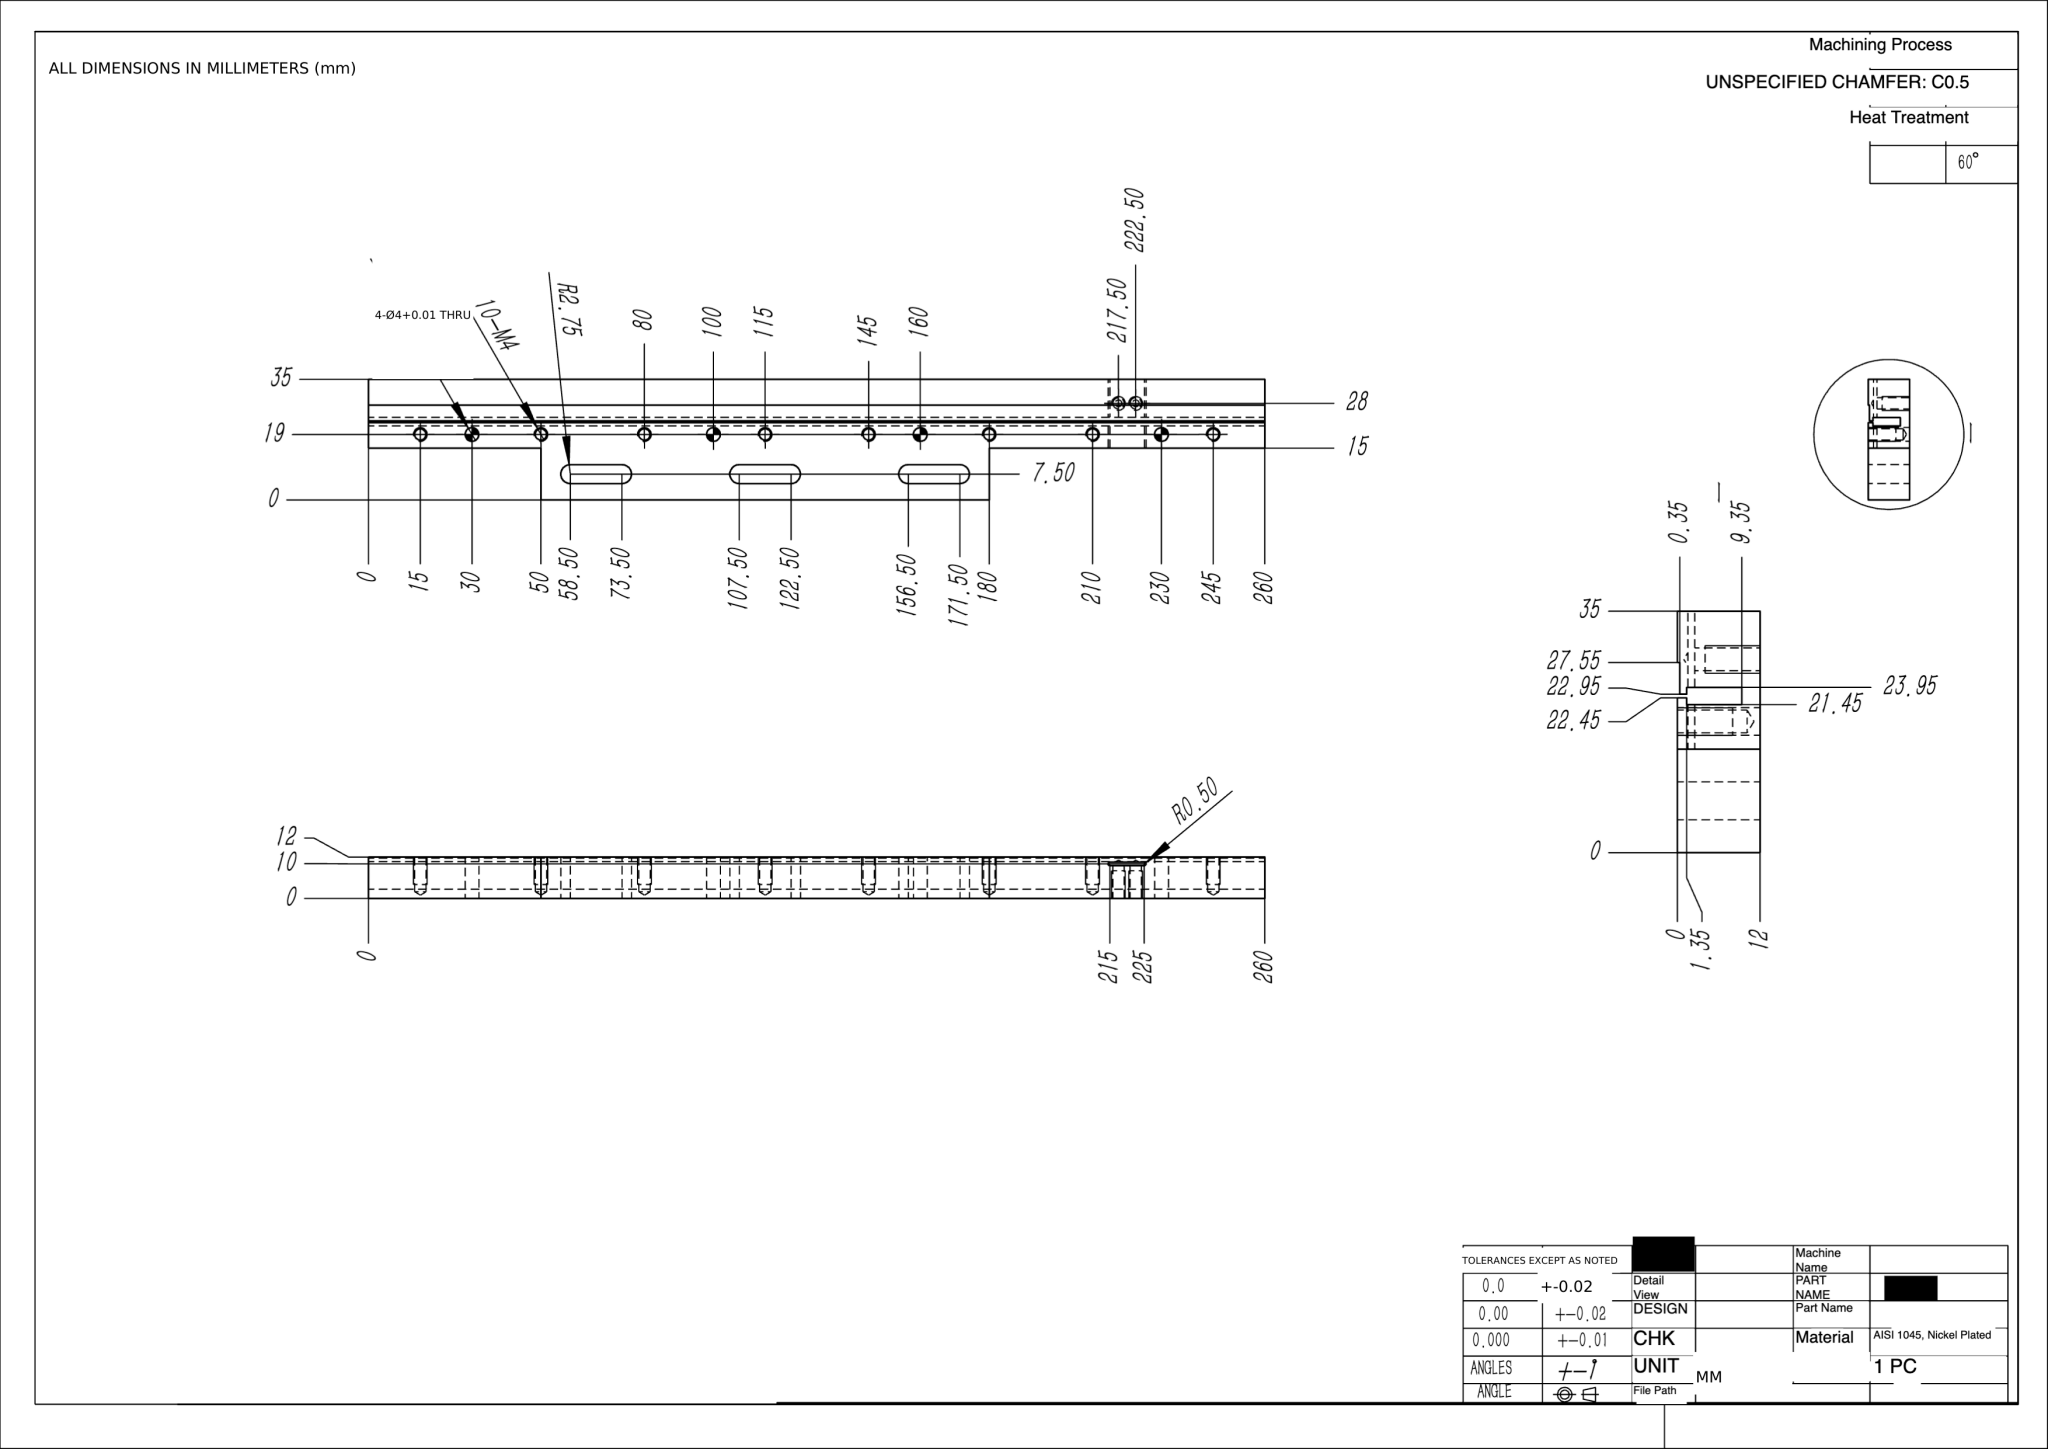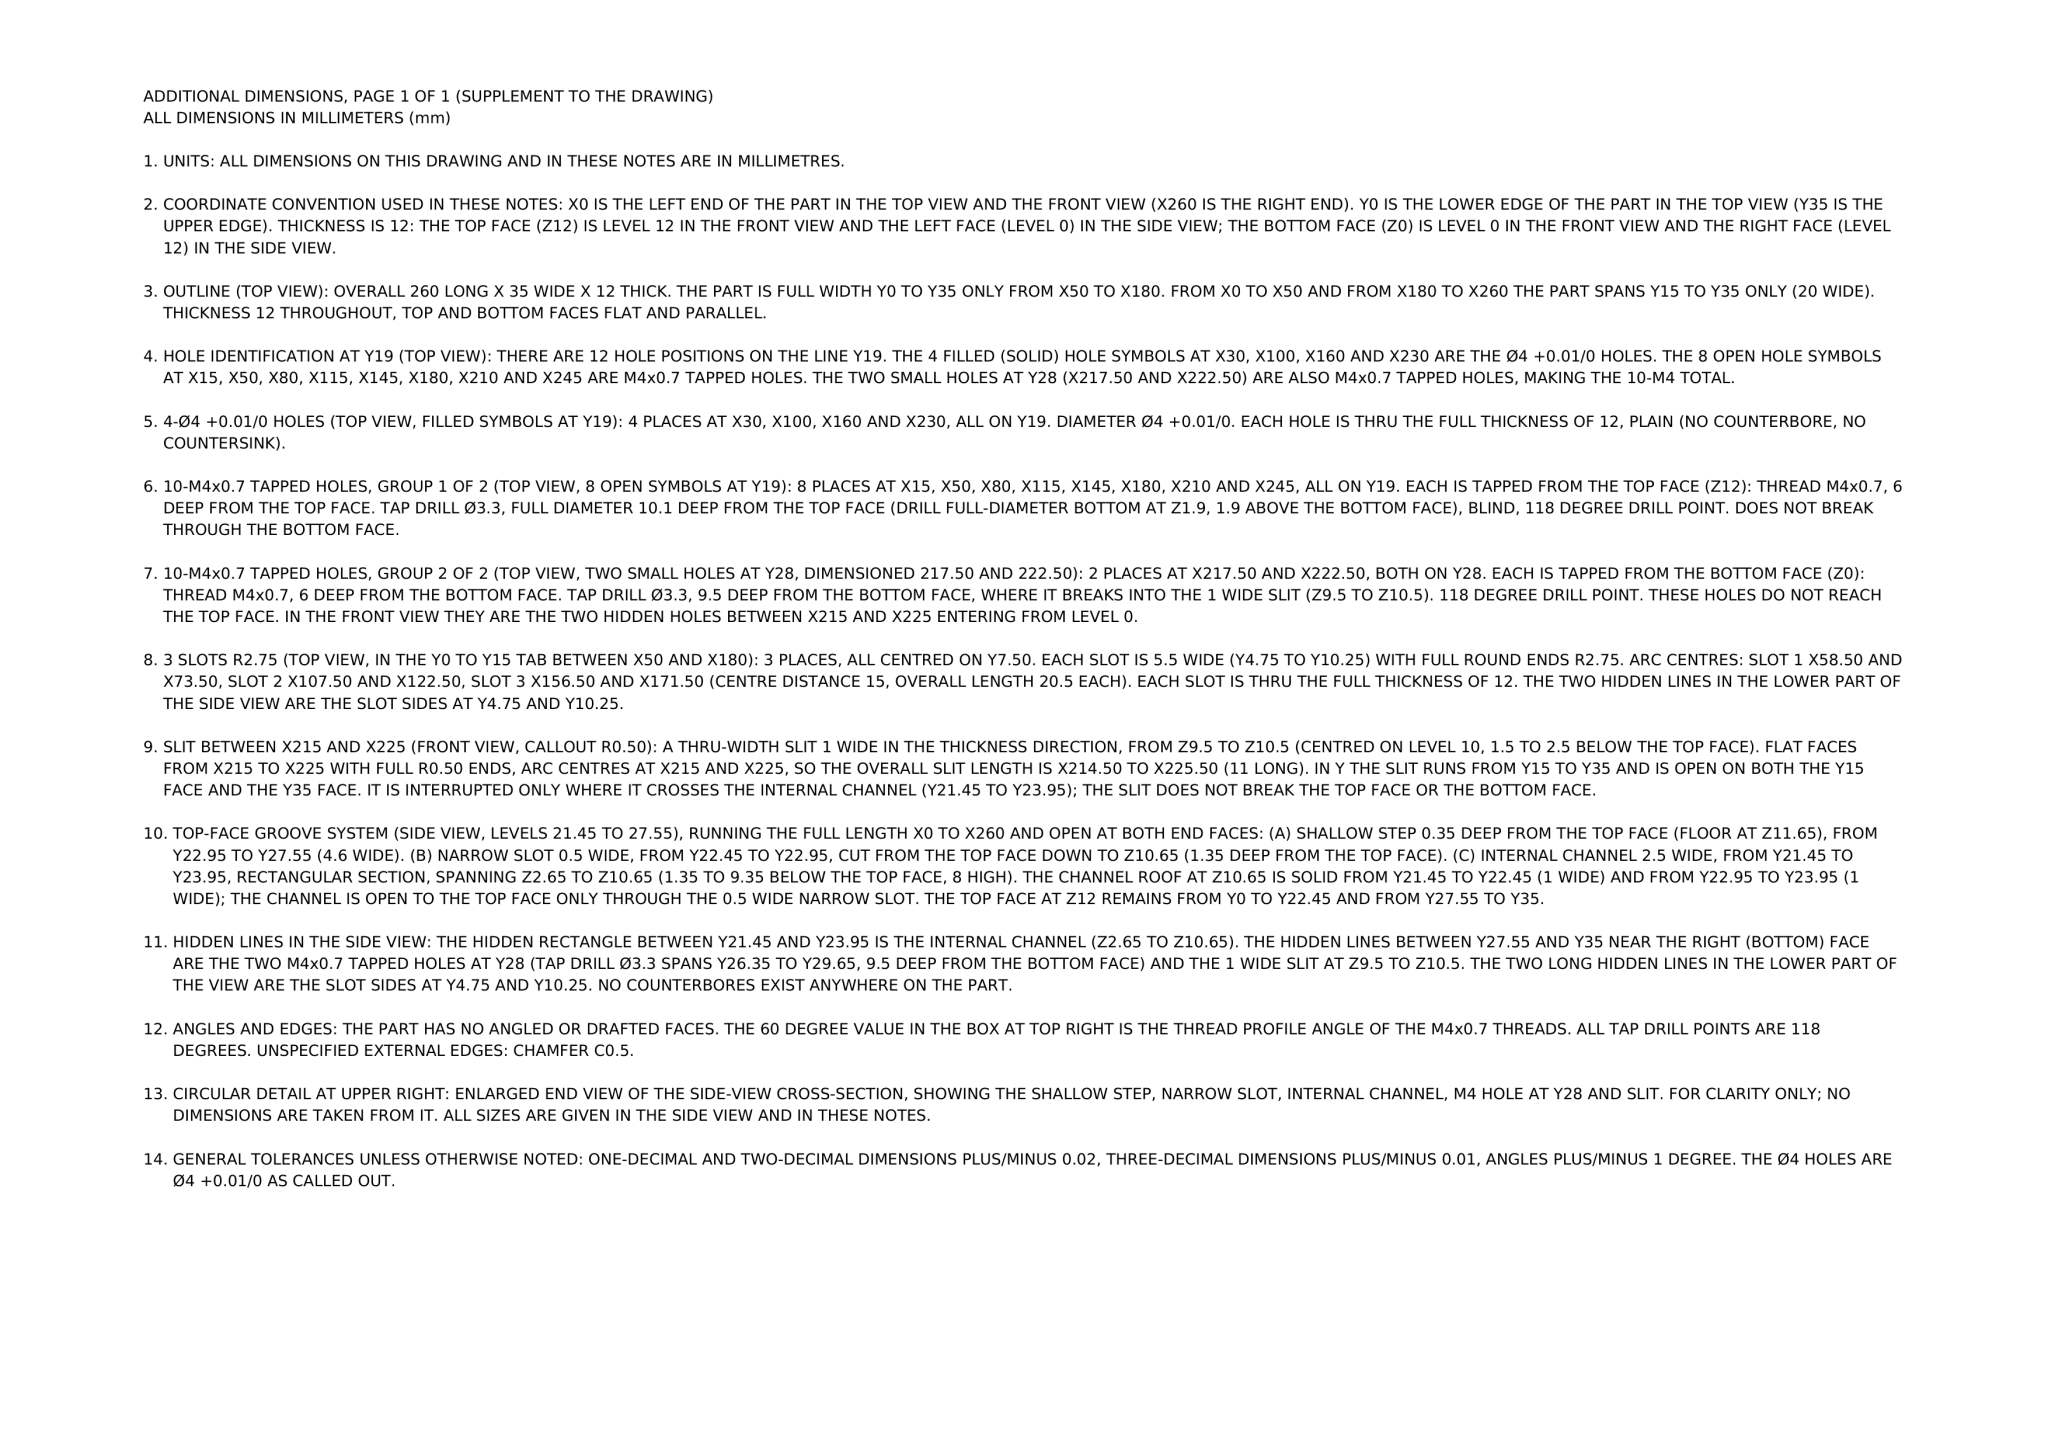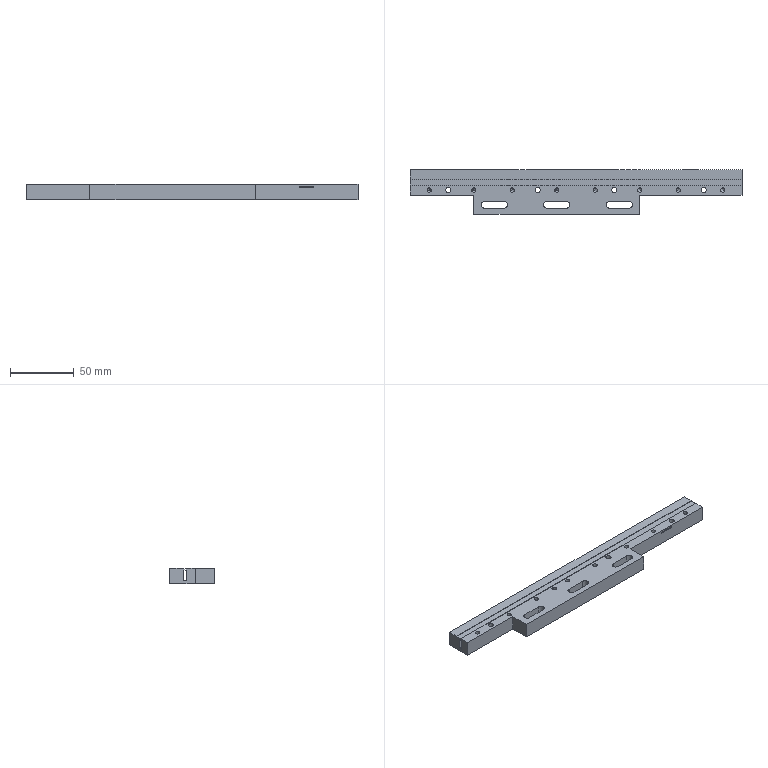Part | NX | mm | 1 solid | 91 faces | box 260 x 35 x 12 mm | volume 74511 mm3 | cylinder 41 | plane 30 | cone 20 | commonest cylinder face diameters 3.3 x20 5.5 x9 4 x8 1 x4